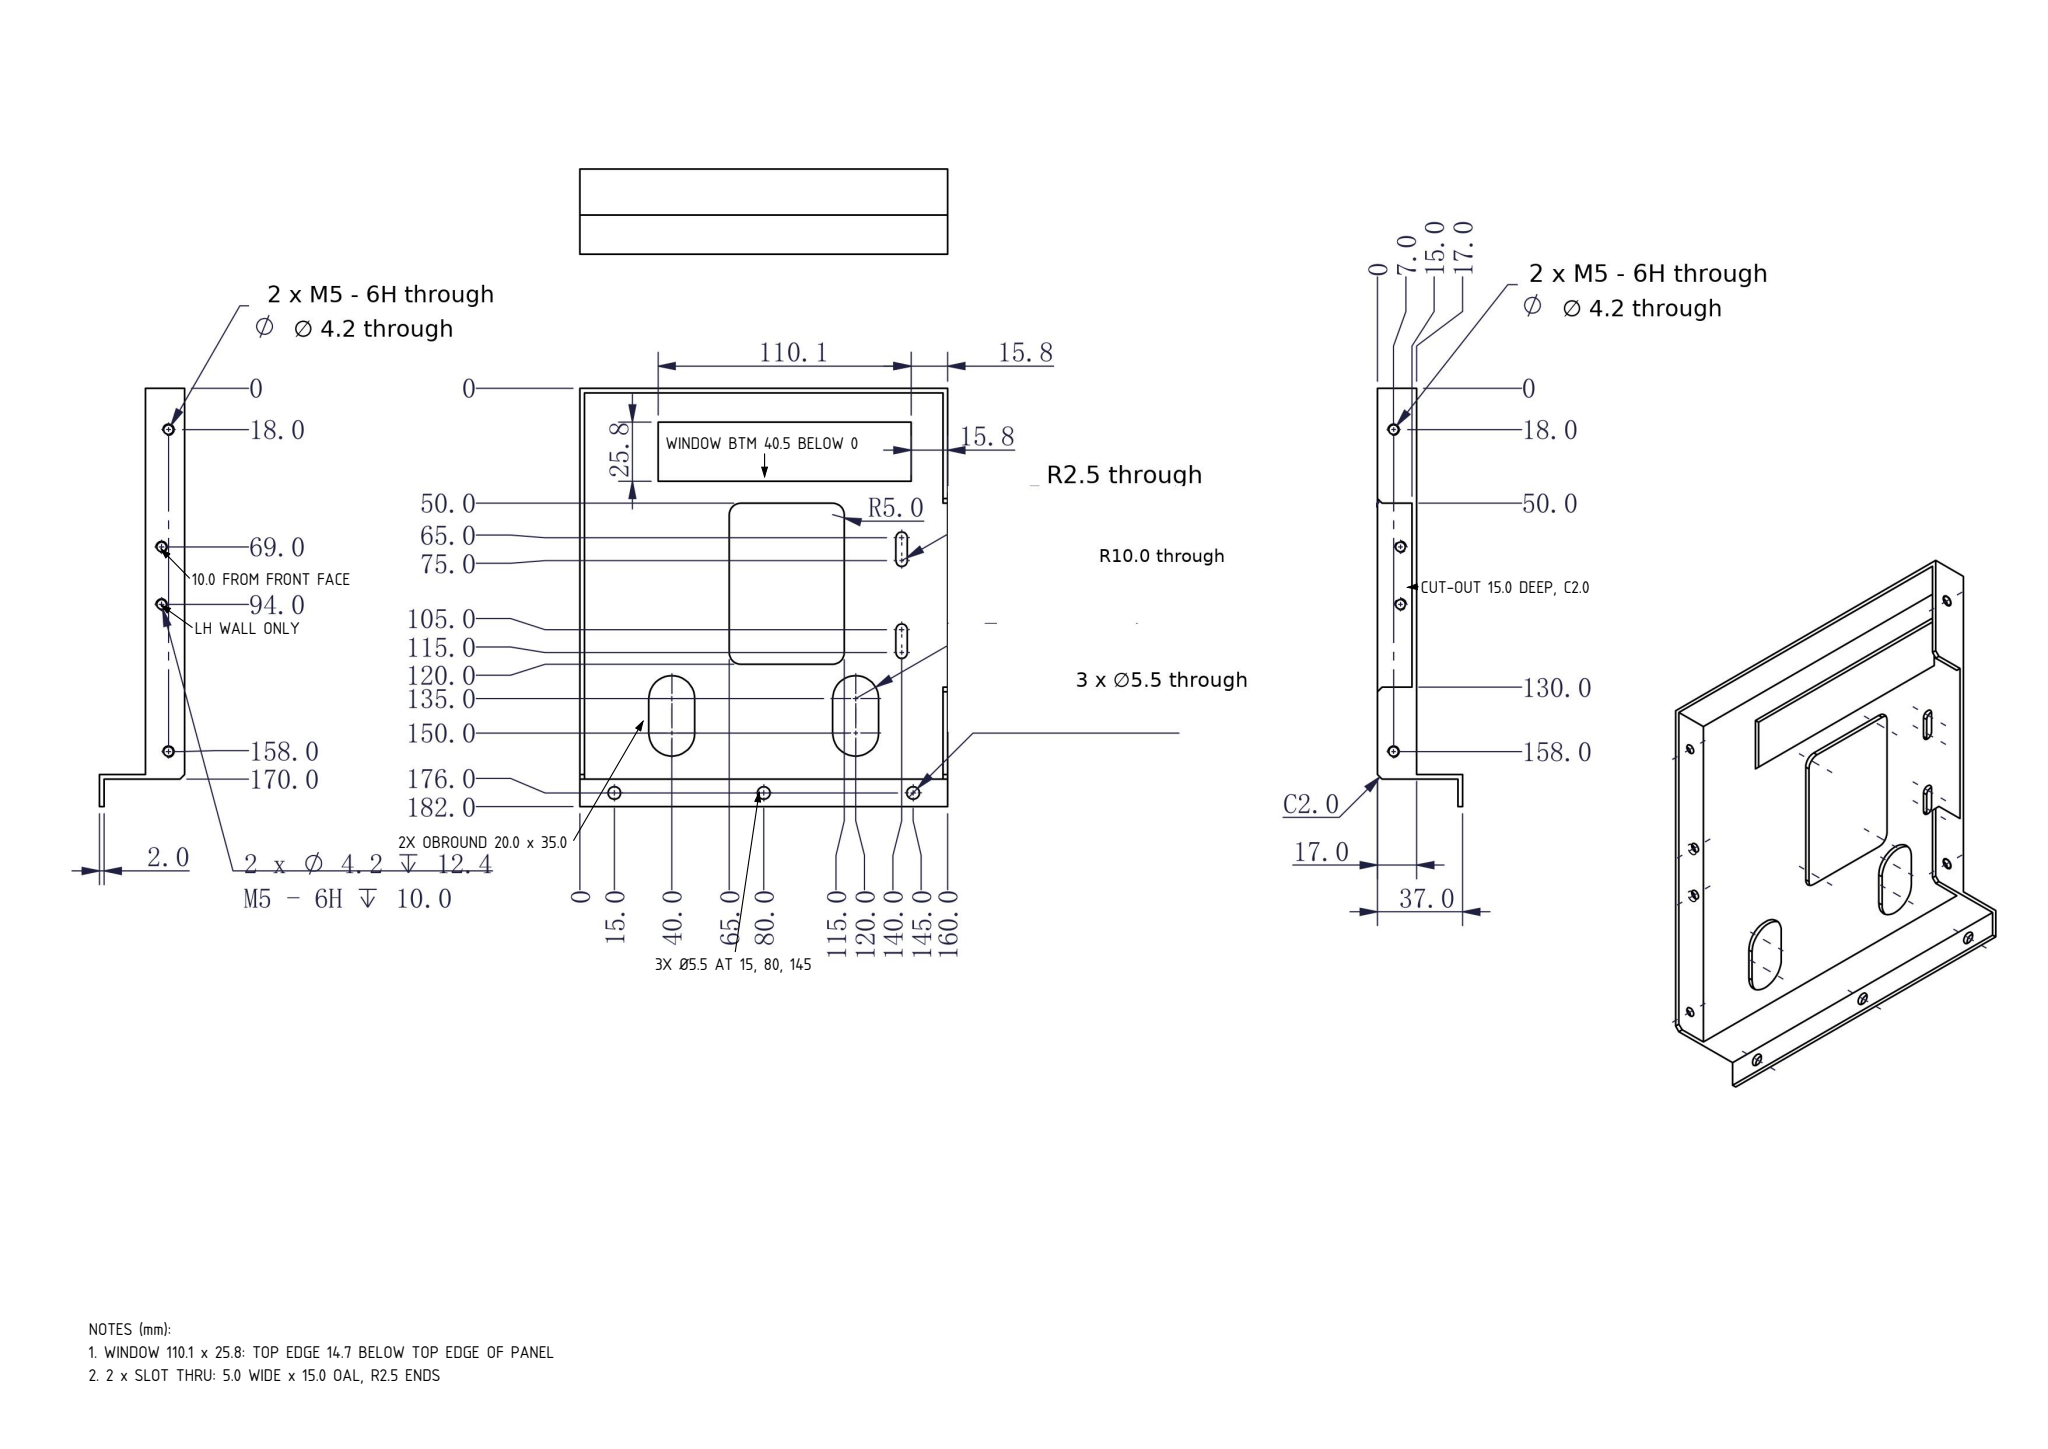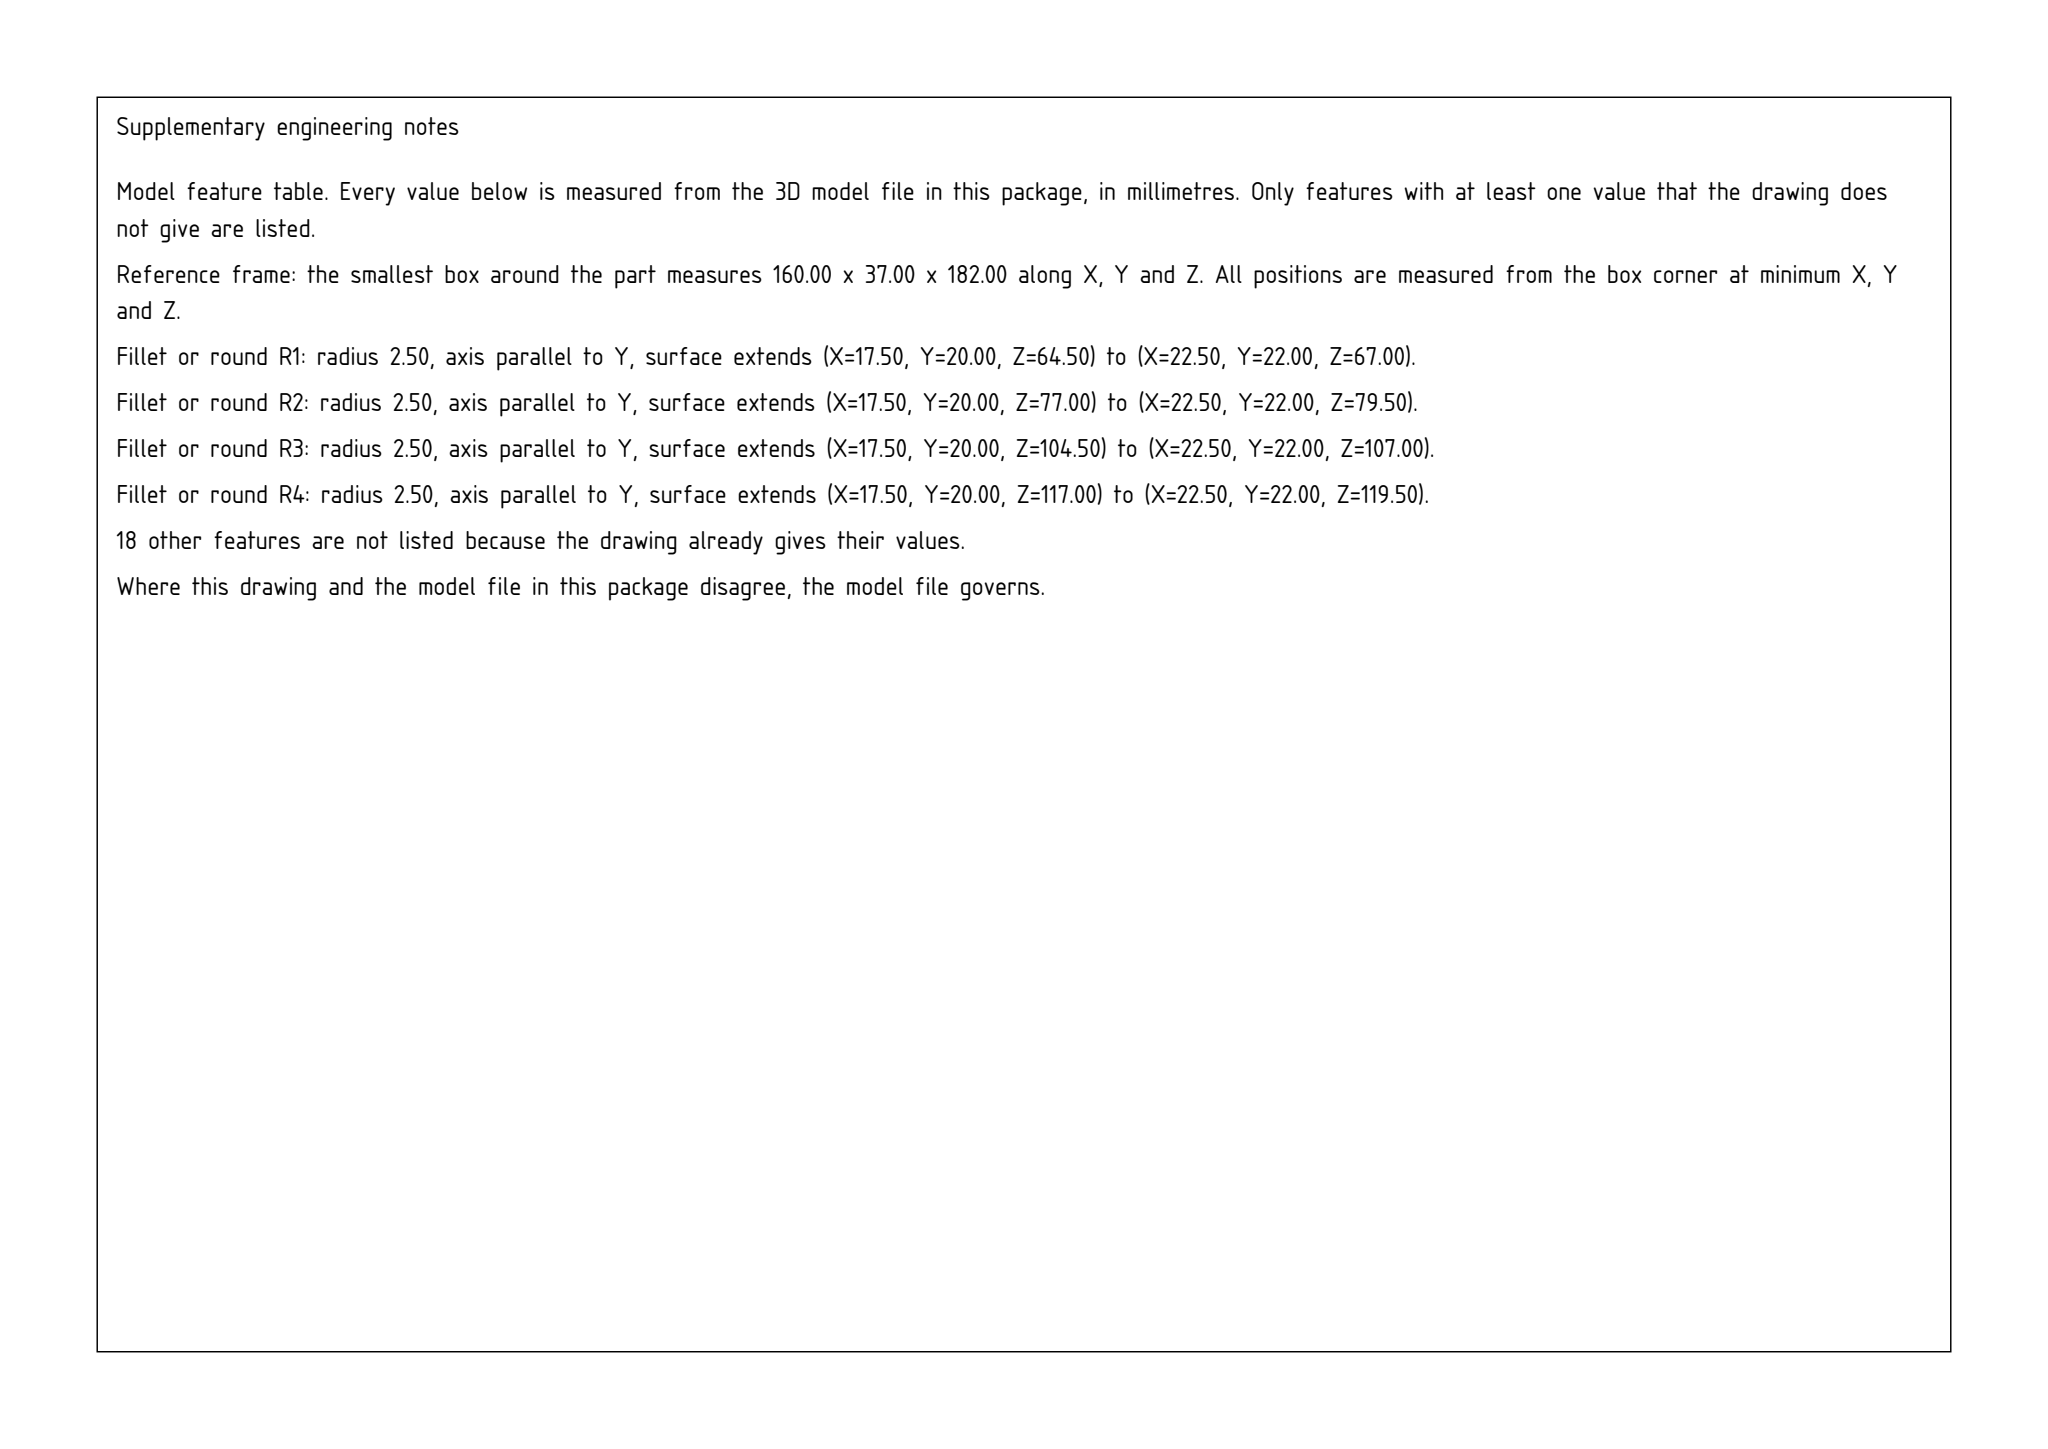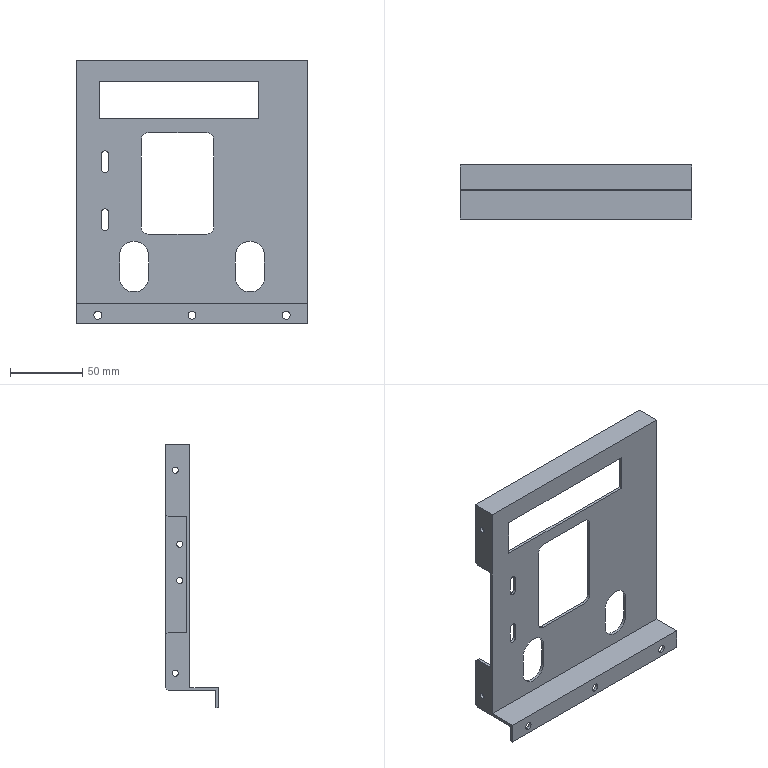Part | SolidWorks | mm | 1 solid | 72 faces | box 160 x 37 x 182 mm | volume 61425 mm3 | plane 38 | cylinder 34 | commonest cylinder face diameters 4.2 x12 20 x6 5 x6 5.5 x6 10 x4
Drawing notes:
TOP WINDOW 110.1 x 25.8: TOP EDGE 14.7, BTM 40.5 BELOW 0 (Z DATUM) | from the solid: z planes 167.28 & 141.5 (182-167.28=14.7, 182-141.5=40.5, diff 25.8); x 15.85/125.96 = 110.1 wide
WINDOW 110.1 x 25.8: TOP EDGE 14.7 BELOW TOP EDGE OF PANEL | from the solid: Window faces z=167.3 & z=141.5 (x 15.8-126.0); panel top z=182 -> 182-167.3=14.7, 167.3-141.5=25.8
SIDE VIEW: HOLES AT 69.0 & 94.0 ARE 10.0 FROM 0 DATUM (FRONT FACE) | from the solid: Ø4.2 holes axis y=27.0 at z=113 & z=88 (x 158-160); front face y=37 -> 37-27=10.0
RH WALL CUT-OUT 50.0 TO 130.0: FULL 15.0 DEEP TO PANEL FACE, C2.0 | from the solid: Wall x=0-2 inner face y22-37 only z12-52 & z132-180; step floors z=52/132 y22-35 + 2x2 chamfers at y35, z50/132
2 x Ø4.2 DP 12.4, M5-6H DP 10.0 AT 69.0 / 94.0: LH WALL ONLY | from the solid: Ø4.2 holes at z=113 & z=88 exist only in wall x 158-160; wall x 0-2 has holes only at z=164 & z=24
2 x OBROUND THRU: 20.0 WIDE x 35.0 OAL, R10.0 ENDS | from the solid: Ø20 arcs at (x40,z32)(x40,z47)(x120,z32)(x120,z47), sides x30/50 & x110/130, y20-22
2 x SLOT THRU: 5.0 WIDE x 15.0 OAL, R2.5 ENDS | from the solid: Ø5 arcs at (x20,z67)(x20,z77)(x20,z107)(x20,z117), sides x=17.5 & 22.5, y20-22
3 x Ø5.5 THRU IN BOTTOM FLANGE AT 15.0, 80.0 & 145.0 | from the solid: Ø5.5 holes axis y, from y0 to y2 (flange), at x=15, 80, 145, z=6
build123d program:
from build123d import *

# Parameters (mm, degrees)
EXTRUDE_THIN1_DEPTH            = 80
F_5_5_5_5_DIAMETER_HOLE1_D     = 5.5
F_5_5_5_5_DIAMETER_HOLE1_DEPTH = 5
F_5_5_5_5_DIAMETER_HOLE1_TIP   = 1.652
CUT_EXTRUDE1_DEPTH             = 10
SKETCH5_W                      = 2
SKETCH5_H                      = 15
BOSS_EXTRUDE1_DEPTH            = 170
SKETCH7_W                      = 80
SKETCH7_H                      = 15
CUT_EXTRUDE2_DEPTH             = 10
SKETCH8_W                      = 160
SKETCH8_H                      = 17
BOSS_EXTRUDE2_DEPTH            = 2
CUT_EXTRUDE3_DEPTH             = 10
CHAMFER1_SIZE                  = 2
CHAMFER2_SIZE                  = 2
M5_TAPPED_HOLE1_D              = 4.2
LPATTERN1_COUNT                = 2
LPATTERN1_PITCH                = 140
CUT_EXTRUDE4_DEPTH             = 10
M5_TAPPED_HOLE2_D              = 4.2
M5_TAPPED_HOLE2_DEPTH          = 12.4
M5_TAPPED_HOLE2_TIP            = 1.262
SKETCH15_W                     = 110.116
SKETCH15_H                     = 25.78
CUT_EXTRUDE5_DEPTH             = 43


with BuildPart() as part:
    # Sketch1 → Extrude-Thin1 (new, symmetric)
    with BuildSketch(Plane(origin=(0, 0, 0), x_dir=(0, 0, -1), z_dir=(1, 0, 0))):
        Polygon((-170, 0), (0, 0), (0, -20), (12, -20), (12, -22), (-2, -22), (-2, -2), (-170, -2), align=None)
    extrude(amount=EXTRUDE_THIN1_DEPTH, both=True)

    # 5.5 _5.5_ Diameter Hole1
    with Locations(Plane(origin=(0, -20, 0), x_dir=(1, 0, 0), z_dir=(0, 1, 0))):
        with Locations((0, 6), (65, 6), (-65, 6)):
            Hole(F_5_5_5_5_DIAMETER_HOLE1_D / 2, depth=F_5_5_5_5_DIAMETER_HOLE1_DEPTH)
            with Locations((0, 0, -(F_5_5_5_5_DIAMETER_HOLE1_DEPTH + F_5_5_5_5_DIAMETER_HOLE1_TIP / 2))):  # 118° drill point
                Cone(0, F_5_5_5_5_DIAMETER_HOLE1_D / 2, F_5_5_5_5_DIAMETER_HOLE1_TIP, mode=Mode.SUBTRACT)

    # Sketch4 → Cut-Extrude1 (cut)
    with BuildSketch(Plane(origin=(0, 0, 0), x_dir=(1, 0, 0), z_dir=(0, 1, 0))):
        with BuildLine():
            Line((-57.5, -55), (-57.5, -65))
            ThreePointArc((-57.5, -65), (-60, -67.5), (-62.5, -65))
            Line((-62.5, -65), (-62.5, -55))
            ThreePointArc((-62.5, -55), (-60, -52.5), (-57.5, -55))
        make_face()
        with BuildLine():
            Line((-57.5, -105), (-57.5, -95))
            ThreePointArc((-57.5, -95), (-60, -92.5), (-62.5, -95))
            Line((-62.5, -95), (-62.5, -105))
            ThreePointArc((-62.5, -105), (-60, -107.5), (-57.5, -105))
        make_face()
    extrude(amount=-CUT_EXTRUDE1_DEPTH, mode=Mode.SUBTRACT)

    # Sketch5 → Boss-Extrude1 (add)
    with BuildSketch(Plane.XY.offset(170)):
        with Locations((79, 7.5)):
            Rectangle(SKETCH5_W, SKETCH5_H)
        with Locations((-79, 7.5)):
            Rectangle(SKETCH5_W, SKETCH5_H)
    extrude(amount=-BOSS_EXTRUDE1_DEPTH)

    # Sketch7 → Cut-Extrude2 (cut)
    with BuildSketch(Plane.ZY.offset(80)):
        with Locations((80, 7.5)):
            Rectangle(SKETCH7_W, SKETCH7_H)
    extrude(amount=-CUT_EXTRUDE2_DEPTH, mode=Mode.SUBTRACT)

    # Sketch8 → Boss-Extrude2 (add)
    with BuildSketch(Plane.XY.offset(170)):
        with Locations((0, 6.5)):
            Rectangle(SKETCH8_W, SKETCH8_H)
    extrude(amount=-BOSS_EXTRUDE2_DEPTH)

    # Sketch9 → Cut-Extrude3 (cut)
    with BuildSketch(Plane(origin=(0, 0, 0), x_dir=(1, 0, 0), z_dir=(0, 1, 0))):
        with BuildLine():
            Line((-50, -35), (-50, -20))
            ThreePointArc((-50, -20), (-40, -10), (-30, -20))
            Line((-30, -20), (-30, -35))
            ThreePointArc((-30, -35), (-40, -45), (-50, -35))
        make_face()
    cut_extrude3 = extrude(amount=-CUT_EXTRUDE3_DEPTH, mode=Mode.SUBTRACT)

    # Mirror2: Cut-Extrude3 across plane
    add(cut_extrude3.mirror(Plane(origin=(0, 0, 0), x_dir=(0, 0, 1), z_dir=(1, 0, 0))), mode=Mode.SUBTRACT)

    # Chamfer1
    chamfer1_edges = [part.edges().sort_by_distance(p)[0] for p in [
        (79, 15, 0),
        (-79, 15, 0),
    ]]
    chamfer(chamfer1_edges, length=CHAMFER1_SIZE)

    # Chamfer2
    chamfer2_edges = [part.edges().sort_by_distance(p)[0] for p in [
        (-79, 15, 120),
        (-79, 15, 40),
    ]]
    chamfer(chamfer2_edges, length=CHAMFER2_SIZE)

    # M5 Tapped Hole1 (through all)
    with Locations(Plane.ZY.offset(80)):
        with Locations((152, 8)):
            m5_tapped_hole1 = Hole(M5_TAPPED_HOLE1_D / 2)

    # LPattern1: M5 Tapped Hole1 ×2
    with Locations(*[(0, 0, -i * LPATTERN1_PITCH) for i in range(1, LPATTERN1_COUNT)]):
        add(m5_tapped_hole1, mode=Mode.SUBTRACT)

    # Sketch12 → Cut-Extrude4 (cut)
    with BuildSketch(Plane.XZ.offset(2)):
        with BuildLine():
            Line((-30, 50), (10, 50))
            ThreePointArc((10, 50), (13.536, 51.464), (15, 55))
            Line((15, 55), (15, 115))
            ThreePointArc((15, 115), (13.536, 118.536), (10, 120))
            Line((10, 120), (-30, 120))
            ThreePointArc((-30, 120), (-33.536, 118.536), (-35, 115))
            Line((-35, 115), (-35, 55))
            ThreePointArc((-35, 55), (-33.536, 51.464), (-30, 50))
        make_face()
    extrude(amount=-CUT_EXTRUDE4_DEPTH, mode=Mode.SUBTRACT)

    # M5 Tapped Hole2
    with Locations(Plane(origin=(80, 0, 0), x_dir=(0, 0, -1), z_dir=(1, 0, 0))):
        with Locations((-101, 5), (-76, 5)):
            Hole(M5_TAPPED_HOLE2_D / 2, depth=M5_TAPPED_HOLE2_DEPTH)
            with Locations((0, 0, -(M5_TAPPED_HOLE2_DEPTH + M5_TAPPED_HOLE2_TIP / 2))):  # 118° drill point
                Cone(0, M5_TAPPED_HOLE2_D / 2, M5_TAPPED_HOLE2_TIP, mode=Mode.SUBTRACT)

    # Sketch15 → Cut-Extrude5 (cut)
    with BuildSketch(Plane(origin=(0, 0, 0), x_dir=(1, 0, 0), z_dir=(0, 1, 0))):
        with Locations((-9.094, -142.391)):
            Rectangle(SKETCH15_W, SKETCH15_H)
    extrude(amount=-CUT_EXTRUDE5_DEPTH, mode=Mode.SUBTRACT)


solid = part.part